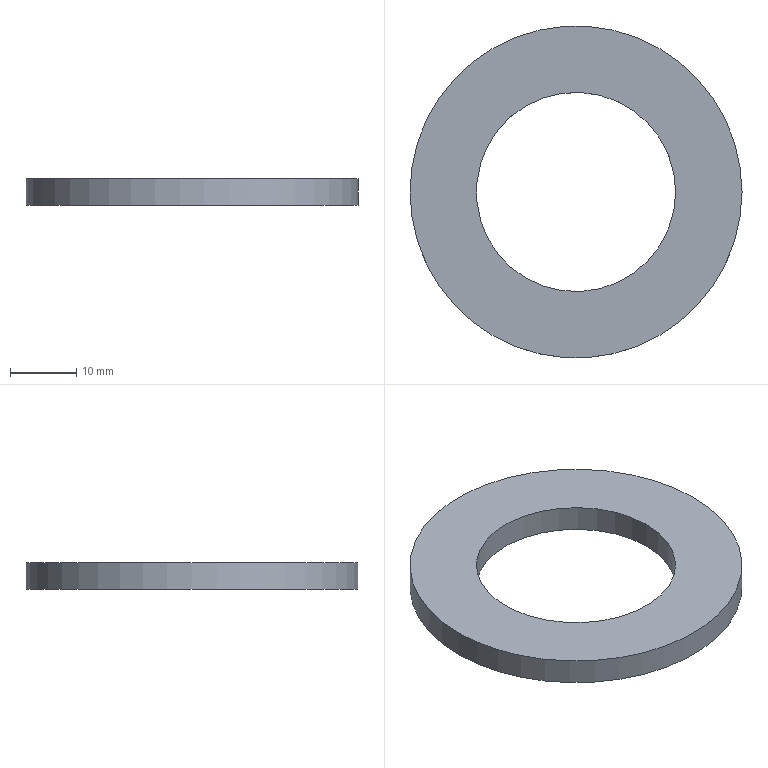Component | NX | GB-T95-2002_M27 | 1 solid | 4 faces | box 50 x 50 x 4 mm | volume 5027 mm3 | cylinder 2 | plane 2 | commonest cylinder face diameters 50 x1 30 x1
STEP:
#1=CARTESIAN_POINT('',(0.,0.,0.));
#2=DIRECTION('',(0.,0.,1.));
#3=DIRECTION('',(1.,0.,0.));
#4=AXIS2_PLACEMENT_3D('',#1,#2,#3);
#5=CARTESIAN_POINT('',(25.,0.,-4.));
#6=VERTEX_POINT('',#5);
#7=CARTESIAN_POINT('',(0.,0.,-4.));
#8=DIRECTION('',(0.,0.,1.));
#9=DIRECTION('',(1.,0.,0.));
#10=AXIS2_PLACEMENT_3D('',#7,#8,#9);
#11=CIRCLE('',#10,25.);
#12=CARTESIAN_POINT('',(0.,0.,0.));
#13=DIRECTION('',(0.,0.,1.));
#14=DIRECTION('',(1.,0.,0.));
#15=AXIS2_PLACEMENT_3D('',#12,#13,#14);
#16=CYLINDRICAL_SURFACE('',#15,25.);
#17=CARTESIAN_POINT('',(0.,-4.));
#18=DIRECTION('',(1.,0.));
#19=VECTOR('',#18,1.);
#20=LINE('',#17,#19);
#21=(GEOMETRIC_REPRESENTATION_CONTEXT(2)PARAMETRIC_REPRESENTATION_CONTEXT()REPRESENTATION_CONTEXT('',''));
#22=DEFINITIONAL_REPRESENTATION('',(#20),#21);
#23=PCURVE('',#16,#22);
#24=CARTESIAN_POINT('',(-25.,0.,-4.));
#25=DIRECTION('',(0.,0.,-1.));
#26=DIRECTION('',(-1.,0.,0.));
#27=AXIS2_PLACEMENT_3D('',#24,#25,#26);
#28=PLANE('',#27);
#29=CARTESIAN_POINT('',(-50.,0.));
#30=CARTESIAN_POINT('',(-50.,43.301));
#31=CARTESIAN_POINT('',(-12.5,21.651));
#32=CARTESIAN_POINT('',(25.,0.));
#33=CARTESIAN_POINT('',(-12.5,-21.651));
#34=CARTESIAN_POINT('',(-50.,-43.301));
#35=CARTESIAN_POINT('',(-50.,0.));
#36=(BOUNDED_CURVE()B_SPLINE_CURVE(2,(#29,#30,#31,#32,#33,#34,#35),.UNSPECIFIED.,.T.,.F.)B_SPLINE_CURVE_WITH_KNOTS((1,2,2,2,2,1),(-2.094,0.,2.094,4.189,6.283,8.378),.UNSPECIFIED.)CURVE()GEOMETRIC_REPRESENTATION_ITEM()RATIONAL_B_SPLINE_CURVE((1.,0.5,1.,0.5,1.,0.5,1.))REPRESENTATION_ITEM(''));
#37=(GEOMETRIC_REPRESENTATION_CONTEXT(2)PARAMETRIC_REPRESENTATION_CONTEXT()REPRESENTATION_CONTEXT('',''));
#38=DEFINITIONAL_REPRESENTATION('',(#36),#37);
#39=PCURVE('',#28,#38);
#40=SURFACE_CURVE('',#11,(#23,#39),.PCURVE_S1.);
#41=EDGE_CURVE('',#6,#6,#40,.T.);
#42=ORIENTED_EDGE('',*,*,#41,.T.);
#43=CARTESIAN_POINT('',(25.,0.,-0.));
#44=VERTEX_POINT('',#43);
#45=CARTESIAN_POINT('',(25.,0.,-4.));
#46=CARTESIAN_POINT('',(25.,0.,-0.));
#47=B_SPLINE_CURVE_WITH_KNOTS('',1,(#45,#46),.UNSPECIFIED.,.F.,.F.,(2,2),(-4.,-0.),.PIECEWISE_BEZIER_KNOTS.);
#48=CARTESIAN_POINT('',(6.283,0.));
#49=DIRECTION('',(0.,1.));
#50=VECTOR('',#49,1.);
#51=LINE('',#48,#50);
#52=(GEOMETRIC_REPRESENTATION_CONTEXT(2)PARAMETRIC_REPRESENTATION_CONTEXT()REPRESENTATION_CONTEXT('',''));
#53=DEFINITIONAL_REPRESENTATION('',(#51),#52);
#54=PCURVE('',#16,#53);
#55=CARTESIAN_POINT('',(0.,0.));
#56=DIRECTION('',(0.,1.));
#57=VECTOR('',#56,1.);
#58=LINE('',#55,#57);
#59=(GEOMETRIC_REPRESENTATION_CONTEXT(2)PARAMETRIC_REPRESENTATION_CONTEXT()REPRESENTATION_CONTEXT('',''));
#60=DEFINITIONAL_REPRESENTATION('',(#58),#59);
#61=PCURVE('',#16,#60);
#62=SEAM_CURVE('',#47,(#54,#61),.PCURVE_S1.);
#63=EDGE_CURVE('',#6,#44,#62,.T.);
#64=ORIENTED_EDGE('',*,*,#63,.T.);
#65=CARTESIAN_POINT('',(0.,0.,-0.));
#66=DIRECTION('',(0.,0.,1.));
#67=DIRECTION('',(1.,0.,0.));
#68=AXIS2_PLACEMENT_3D('',#65,#66,#67);
#69=CIRCLE('',#68,25.);
#70=CARTESIAN_POINT('',(0.,-0.));
#71=DIRECTION('',(1.,0.));
#72=VECTOR('',#71,1.);
#73=LINE('',#70,#72);
#74=(GEOMETRIC_REPRESENTATION_CONTEXT(2)PARAMETRIC_REPRESENTATION_CONTEXT()REPRESENTATION_CONTEXT('',''));
#75=DEFINITIONAL_REPRESENTATION('',(#73),#74);
#76=PCURVE('',#16,#75);
#77=CARTESIAN_POINT('',(-15.,0.,-0.));
#78=DIRECTION('',(0.,0.,1.));
#79=DIRECTION('',(1.,0.,0.));
#80=AXIS2_PLACEMENT_3D('',#77,#78,#79);
#81=PLANE('',#80);
#82=CARTESIAN_POINT('',(15.,0.));
#83=DIRECTION('',(1.,0.));
#84=AXIS2_PLACEMENT_2D('',#82,#83);
#85=CIRCLE('',#84,25.);
#86=(GEOMETRIC_REPRESENTATION_CONTEXT(2)PARAMETRIC_REPRESENTATION_CONTEXT()REPRESENTATION_CONTEXT('',''));
#87=DEFINITIONAL_REPRESENTATION('',(#85),#86);
#88=PCURVE('',#81,#87);
#89=SURFACE_CURVE('',#69,(#76,#88),.PCURVE_S1.);
#90=EDGE_CURVE('',#44,#44,#89,.T.);
#91=ORIENTED_EDGE('',*,*,#90,.F.);
#92=ORIENTED_EDGE('',*,*,#63,.F.);
#93=EDGE_LOOP('',(#42,#64,#91,#92));
#94=FACE_BOUND('',#93,.T.);
#95=ADVANCED_FACE('',(#94),#16,.T.);
#96=CARTESIAN_POINT('',(15.,0.,-4.));
#97=VERTEX_POINT('',#96);
#98=CARTESIAN_POINT('',(0.,0.,-4.));
#99=DIRECTION('',(0.,0.,1.));
#100=DIRECTION('',(1.,0.,0.));
#101=AXIS2_PLACEMENT_3D('',#98,#99,#100);
#102=CIRCLE('',#101,15.);
#103=CARTESIAN_POINT('',(-40.,0.));
#104=CARTESIAN_POINT('',(-40.,25.981));
#105=CARTESIAN_POINT('',(-17.5,12.99));
#106=CARTESIAN_POINT('',(5.,0.));
#107=CARTESIAN_POINT('',(-17.5,-12.99));
#108=CARTESIAN_POINT('',(-40.,-25.981));
#109=CARTESIAN_POINT('',(-40.,0.));
#110=(BOUNDED_CURVE()B_SPLINE_CURVE(2,(#103,#104,#105,#106,#107,#108,#109),.UNSPECIFIED.,.T.,.F.)B_SPLINE_CURVE_WITH_KNOTS((1,2,2,2,2,1),(-2.094,0.,2.094,4.189,6.283,8.378),.UNSPECIFIED.)CURVE()GEOMETRIC_REPRESENTATION_ITEM()RATIONAL_B_SPLINE_CURVE((1.,0.5,1.,0.5,1.,0.5,1.))REPRESENTATION_ITEM(''));
#111=(GEOMETRIC_REPRESENTATION_CONTEXT(2)PARAMETRIC_REPRESENTATION_CONTEXT()REPRESENTATION_CONTEXT('',''));
#112=DEFINITIONAL_REPRESENTATION('',(#110),#111);
#113=PCURVE('',#28,#112);
#114=CARTESIAN_POINT('',(0.,0.,0.));
#115=DIRECTION('',(0.,0.,1.));
#116=DIRECTION('',(1.,0.,0.));
#117=AXIS2_PLACEMENT_3D('',#114,#115,#116);
#118=CYLINDRICAL_SURFACE('',#117,15.);
#119=CARTESIAN_POINT('',(0.,-4.));
#120=DIRECTION('',(1.,0.));
#121=VECTOR('',#120,1.);
#122=LINE('',#119,#121);
#123=(GEOMETRIC_REPRESENTATION_CONTEXT(2)PARAMETRIC_REPRESENTATION_CONTEXT()REPRESENTATION_CONTEXT('',''));
#124=DEFINITIONAL_REPRESENTATION('',(#122),#123);
#125=PCURVE('',#118,#124);
#126=SURFACE_CURVE('',#102,(#113,#125),.PCURVE_S1.);
#127=EDGE_CURVE('',#97,#97,#126,.T.);
#128=ORIENTED_EDGE('',*,*,#127,.T.);
#129=EDGE_LOOP('',(#128));
#130=FACE_BOUND('',#129,.T.);
#131=ORIENTED_EDGE('',*,*,#41,.F.);
#132=EDGE_LOOP('',(#131));
#133=FACE_BOUND('',#132,.T.);
#134=ADVANCED_FACE('',(#130,#133),#28,.T.);
#135=CARTESIAN_POINT('',(15.,0.,0.));
#136=VERTEX_POINT('',#135);
#137=CARTESIAN_POINT('',(0.,0.,0.));
#138=DIRECTION('',(0.,0.,1.));
#139=DIRECTION('',(1.,0.,0.));
#140=AXIS2_PLACEMENT_3D('',#137,#138,#139);
#141=CIRCLE('',#140,15.);
#142=CARTESIAN_POINT('',(0.,0.));
#143=DIRECTION('',(1.,0.));
#144=VECTOR('',#143,1.);
#145=LINE('',#142,#144);
#146=(GEOMETRIC_REPRESENTATION_CONTEXT(2)PARAMETRIC_REPRESENTATION_CONTEXT()REPRESENTATION_CONTEXT('',''));
#147=DEFINITIONAL_REPRESENTATION('',(#145),#146);
#148=PCURVE('',#118,#147);
#149=CARTESIAN_POINT('',(15.,0.));
#150=DIRECTION('',(1.,0.));
#151=AXIS2_PLACEMENT_2D('',#149,#150);
#152=CIRCLE('',#151,15.);
#153=(GEOMETRIC_REPRESENTATION_CONTEXT(2)PARAMETRIC_REPRESENTATION_CONTEXT()REPRESENTATION_CONTEXT('',''));
#154=DEFINITIONAL_REPRESENTATION('',(#152),#153);
#155=PCURVE('',#81,#154);
#156=SURFACE_CURVE('',#141,(#148,#155),.PCURVE_S1.);
#157=EDGE_CURVE('',#136,#136,#156,.T.);
#158=ORIENTED_EDGE('',*,*,#157,.F.);
#159=CARTESIAN_POINT('',(15.,-0.,-4.));
#160=CARTESIAN_POINT('',(15.,-0.,0.));
#161=B_SPLINE_CURVE_WITH_KNOTS('',1,(#159,#160),.UNSPECIFIED.,.F.,.F.,(2,2),(-4.,0.),.PIECEWISE_BEZIER_KNOTS.);
#162=CARTESIAN_POINT('',(0.,0.));
#163=DIRECTION('',(0.,1.));
#164=VECTOR('',#163,1.);
#165=LINE('',#162,#164);
#166=(GEOMETRIC_REPRESENTATION_CONTEXT(2)PARAMETRIC_REPRESENTATION_CONTEXT()REPRESENTATION_CONTEXT('',''));
#167=DEFINITIONAL_REPRESENTATION('',(#165),#166);
#168=PCURVE('',#118,#167);
#169=CARTESIAN_POINT('',(6.283,0.));
#170=DIRECTION('',(0.,1.));
#171=VECTOR('',#170,1.);
#172=LINE('',#169,#171);
#173=(GEOMETRIC_REPRESENTATION_CONTEXT(2)PARAMETRIC_REPRESENTATION_CONTEXT()REPRESENTATION_CONTEXT('',''));
#174=DEFINITIONAL_REPRESENTATION('',(#172),#173);
#175=PCURVE('',#118,#174);
#176=SEAM_CURVE('',#161,(#168,#175),.PCURVE_S1.);
#177=EDGE_CURVE('',#97,#136,#176,.T.);
#178=ORIENTED_EDGE('',*,*,#177,.F.);
#179=ORIENTED_EDGE('',*,*,#127,.T.);
#180=ORIENTED_EDGE('',*,*,#177,.T.);
#181=EDGE_LOOP('',(#158,#178,#179,#180));
#182=FACE_BOUND('',#181,.F.);
#183=ADVANCED_FACE('',(#182),#118,.F.);
#184=ORIENTED_EDGE('',*,*,#90,.T.);
#185=EDGE_LOOP('',(#184));
#186=FACE_BOUND('',#185,.T.);
#187=ORIENTED_EDGE('',*,*,#157,.F.);
#188=EDGE_LOOP('',(#187));
#189=FACE_BOUND('',#188,.T.);
#190=ADVANCED_FACE('',(#186,#189),#81,.T.);
#191=CLOSED_SHELL('',(#95,#134,#183,#190));
#192=MANIFOLD_SOLID_BREP('',#191);
#193=(LENGTH_UNIT()NAMED_UNIT(*)SI_UNIT(.MILLI.,.METRE.));
#194=UNCERTAINTY_MEASURE_WITH_UNIT(LENGTH_MEASURE(0.00001),#193,'','');
#195=(NAMED_UNIT(*)PLANE_ANGLE_UNIT()SI_UNIT($,.RADIAN.));
#196=(NAMED_UNIT(*)SI_UNIT($,.STERADIAN.)SOLID_ANGLE_UNIT());
#197=(GEOMETRIC_REPRESENTATION_CONTEXT(3)GLOBAL_UNCERTAINTY_ASSIGNED_CONTEXT((#194))GLOBAL_UNIT_ASSIGNED_CONTEXT((#193,#195,#196))REPRESENTATION_CONTEXT('',''));
#198=ADVANCED_BREP_SHAPE_REPRESENTATION('',(#4,#192),#197);